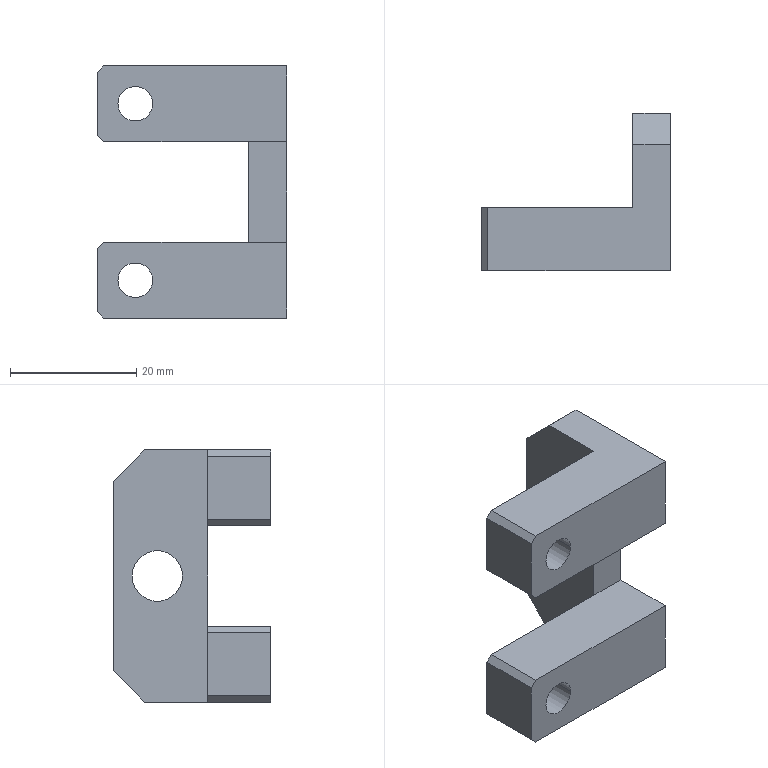Component | SolidWorks | 312981493LimitBlock-1 | 1 solid | 26 faces | box 30 x 25 x 40 mm | volume 9853 mm3 | plane 20 | cylinder 6 | commonest cylinder face diameters 5.5 x4 8 x2 | material Plain Carbon Steel
build123d program:
from build123d import *

# Parameters (mm, degrees)
SKETCH1_W            = 25
SKETCH1_H            = 40
BOSS_EXTRUDE1_DEPTH  = 30
SKETCH5_W            = 15
SKETCH5_H            = 40
CUT_EXTRUDE2_DEPTH   = 24
SKETCH9_W            = 10
SKETCH9_H            = 16
CUT_EXTRUDE4_DEPTH   = 56.902
CHAMFER2_SIZE        = 5
M5_CLEARANCE_HOLE1_D = 5.5
LPATTERN1_COUNT      = 2
LPATTERN1_PITCH      = 28
CHAMFER3_SIZE        = 1
M8_TAPPED_HOLE1_D    = 8


with BuildPart() as part:
    # Sketch1 → Boss-Extrude1 (new body)
    with BuildSketch(Plane.XY):
        with Locations((12.5, 20)):
            Rectangle(SKETCH1_W, SKETCH1_H)
    extrude(amount=BOSS_EXTRUDE1_DEPTH)

    # Sketch5 → Cut-Extrude2 (cut)
    with BuildSketch(Plane.XY.offset(30)):
        with Locations((7.5, 20)):
            Rectangle(SKETCH5_W, SKETCH5_H)
    extrude(amount=-CUT_EXTRUDE2_DEPTH, mode=Mode.SUBTRACT)

    # Sketch9 → Cut-Extrude4 (cut, through all)
    with BuildSketch(Plane.XY.offset(30)):
        with Locations((20, 20)):
            Rectangle(SKETCH9_W, SKETCH9_H)
    extrude(amount=-CUT_EXTRUDE4_DEPTH, mode=Mode.SUBTRACT)

    # Chamfer2
    chamfer2_edges = [part.edges().sort_by_distance(p)[0] for p in [
        (0, 40, 3),
        (0, 0, 3),
    ]]
    chamfer(chamfer2_edges, length=CHAMFER2_SIZE)

    # M5 Clearance Hole1 (through all)
    with Locations(Plane(origin=(15, 28.184, -31.582), x_dir=(0, 0, 1), z_dir=(-1, 0, 0))):
        with Locations((55.582, -22.184)):
            m5_clearance_hole1 = Hole(M5_CLEARANCE_HOLE1_D / 2)

    # LPattern1: M5 Clearance Hole1 ×2
    with Locations(*[(0, i * LPATTERN1_PITCH, 0) for i in range(1, LPATTERN1_COUNT)]):
        add(m5_clearance_hole1, mode=Mode.SUBTRACT)

    # Chamfer3
    chamfer3_edges = [part.edges().sort_by_distance(p)[0] for p in [
        (20, 40, 30),
        (20, 0, 30),
        (20, 28, 30),
        (20, 12, 30),
    ]]
    chamfer(chamfer3_edges, length=CHAMFER3_SIZE)

    # M8 Tapped Hole1 (through all)
    with Locations(Plane.XY.offset(6)):
        with Locations((7, 20)):
            Hole(M8_TAPPED_HOLE1_D / 2)


solid = part.part

# Placed as in the assembly
solid = solid.moved(Location((36.27, 33.768, 18.329), (90, -90, 0)))
STEP:
#1=COLOUR_RGB('',0.7922,0.8196,0.9333);
#2=FILL_AREA_STYLE_COLOUR('',#1);
#3=FILL_AREA_STYLE('',(#2));
#4=SURFACE_STYLE_FILL_AREA(#3);
#5=SURFACE_SIDE_STYLE('',(#4));
#6=SURFACE_STYLE_USAGE(.BOTH.,#5);
#7=PRESENTATION_STYLE_ASSIGNMENT((#6));
#8=CARTESIAN_POINT('',(1.428,1.211,1.509));
#9=VERTEX_POINT('',#8);
#10=CARTESIAN_POINT('',(1.428,0.8964,1.509));
#11=VERTEX_POINT('',#10);
#12=CARTESIAN_POINT('',(1.428,1.054,1.509));
#13=DIRECTION('',(-1.,-0.,-0.));
#14=DIRECTION('',(0.,-1.,0.));
#15=AXIS2_PLACEMENT_3D('',#12,#13,#14);
#16=CIRCLE('',#15,0.1575);
#17=EDGE_CURVE('',#9,#11,#16,.T.);
#18=ORIENTED_EDGE('',*,*,#17,.F.);
#19=CARTESIAN_POINT('',(1.192,1.211,1.509));
#20=VERTEX_POINT('',#19);
#21=CARTESIAN_POINT('',(1.192,1.211,1.509));
#22=DIRECTION('',(-1.,-0.,-0.));
#23=VECTOR('',#22,39.37);
#24=LINE('',#21,#23);
#25=EDGE_CURVE('',#9,#20,#24,.T.);
#26=ORIENTED_EDGE('',*,*,#25,.T.);
#27=CARTESIAN_POINT('',(1.192,0.8964,1.509));
#28=VERTEX_POINT('',#27);
#29=CARTESIAN_POINT('',(1.192,1.054,1.509));
#30=DIRECTION('',(-1.,-0.,-0.));
#31=DIRECTION('',(0.,-1.,0.));
#32=AXIS2_PLACEMENT_3D('',#29,#30,#31);
#33=CIRCLE('',#32,0.1575);
#34=EDGE_CURVE('',#20,#28,#33,.T.);
#35=ORIENTED_EDGE('',*,*,#34,.T.);
#36=CARTESIAN_POINT('',(1.192,0.8964,1.509));
#37=DIRECTION('',(-1.,-0.,-0.));
#38=VECTOR('',#37,39.37);
#39=LINE('',#36,#38);
#40=EDGE_CURVE('',#11,#28,#39,.T.);
#41=ORIENTED_EDGE('',*,*,#40,.F.);
#42=EDGE_LOOP('',(#18,#26,#35,#41));
#43=FACE_OUTER_BOUND('',#42,.T.);
#44=CARTESIAN_POINT('',(1.192,1.054,1.509));
#45=DIRECTION('',(-1.,-0.,-0.));
#46=DIRECTION('',(0.,-1.,0.));
#47=AXIS2_PLACEMENT_3D('',#44,#45,#46);
#48=CYLINDRICAL_SURFACE('',#47,0.1575);
#49=ADVANCED_FACE('',(#43),#48,.F.);
#50=CARTESIAN_POINT('',(0.5913,0.3452,2.06));
#51=VERTEX_POINT('',#50);
#52=CARTESIAN_POINT('',(0.3748,0.3452,2.06));
#53=VERTEX_POINT('',#52);
#54=CARTESIAN_POINT('',(0.4831,0.3452,2.06));
#55=DIRECTION('',(-0.,1.,-0.));
#56=DIRECTION('',(-1.,0.,0.));
#57=AXIS2_PLACEMENT_3D('',#54,#55,#56);
#58=CIRCLE('',#57,0.1083);
#59=EDGE_CURVE('',#51,#53,#58,.T.);
#60=ORIENTED_EDGE('',*,*,#59,.F.);
#61=CARTESIAN_POINT('',(0.5913,0.7389,2.06));
#62=VERTEX_POINT('',#61);
#63=CARTESIAN_POINT('',(0.5913,0.7389,2.06));
#64=DIRECTION('',(-0.,1.,-0.));
#65=VECTOR('',#64,39.37);
#66=LINE('',#63,#65);
#67=EDGE_CURVE('',#51,#62,#66,.T.);
#68=ORIENTED_EDGE('',*,*,#67,.T.);
#69=CARTESIAN_POINT('',(0.3748,0.7389,2.06));
#70=VERTEX_POINT('',#69);
#71=CARTESIAN_POINT('',(0.4831,0.7389,2.06));
#72=DIRECTION('',(-0.,1.,-0.));
#73=DIRECTION('',(-1.,0.,0.));
#74=AXIS2_PLACEMENT_3D('',#71,#72,#73);
#75=CIRCLE('',#74,0.1083);
#76=EDGE_CURVE('',#62,#70,#75,.T.);
#77=ORIENTED_EDGE('',*,*,#76,.T.);
#78=CARTESIAN_POINT('',(0.3748,0.7389,2.06));
#79=DIRECTION('',(-0.,1.,-0.));
#80=VECTOR('',#79,39.37);
#81=LINE('',#78,#80);
#82=EDGE_CURVE('',#53,#70,#81,.T.);
#83=ORIENTED_EDGE('',*,*,#82,.F.);
#84=EDGE_LOOP('',(#60,#68,#77,#83));
#85=FACE_OUTER_BOUND('',#84,.T.);
#86=CARTESIAN_POINT('',(0.4831,0.7389,2.06));
#87=DIRECTION('',(-0.,1.,-0.));
#88=DIRECTION('',(-1.,0.,0.));
#89=AXIS2_PLACEMENT_3D('',#86,#87,#88);
#90=CYLINDRICAL_SURFACE('',#89,0.1083);
#91=ADVANCED_FACE('',(#85),#90,.F.);
#92=CARTESIAN_POINT('',(0.5913,0.3452,0.9579));
#93=VERTEX_POINT('',#92);
#94=CARTESIAN_POINT('',(0.3748,0.3452,0.9579));
#95=VERTEX_POINT('',#94);
#96=CARTESIAN_POINT('',(0.4831,0.3452,0.9579));
#97=DIRECTION('',(-0.,1.,-0.));
#98=DIRECTION('',(-1.,0.,0.));
#99=AXIS2_PLACEMENT_3D('',#96,#97,#98);
#100=CIRCLE('',#99,0.1083);
#101=EDGE_CURVE('',#93,#95,#100,.T.);
#102=ORIENTED_EDGE('',*,*,#101,.F.);
#103=CARTESIAN_POINT('',(0.5913,0.7389,0.9579));
#104=VERTEX_POINT('',#103);
#105=CARTESIAN_POINT('',(0.5913,0.7389,0.9579));
#106=DIRECTION('',(-0.,1.,-0.));
#107=VECTOR('',#106,39.37);
#108=LINE('',#105,#107);
#109=EDGE_CURVE('',#93,#104,#108,.T.);
#110=ORIENTED_EDGE('',*,*,#109,.T.);
#111=CARTESIAN_POINT('',(0.3748,0.7389,0.9579));
#112=VERTEX_POINT('',#111);
#113=CARTESIAN_POINT('',(0.4831,0.7389,0.9579));
#114=DIRECTION('',(-0.,1.,-0.));
#115=DIRECTION('',(-1.,0.,0.));
#116=AXIS2_PLACEMENT_3D('',#113,#114,#115);
#117=CIRCLE('',#116,0.1083);
#118=EDGE_CURVE('',#104,#112,#117,.T.);
#119=ORIENTED_EDGE('',*,*,#118,.T.);
#120=CARTESIAN_POINT('',(0.3748,0.7389,0.9579));
#121=DIRECTION('',(-0.,1.,-0.));
#122=VECTOR('',#121,39.37);
#123=LINE('',#120,#122);
#124=EDGE_CURVE('',#95,#112,#123,.T.);
#125=ORIENTED_EDGE('',*,*,#124,.F.);
#126=EDGE_LOOP('',(#102,#110,#119,#125));
#127=FACE_OUTER_BOUND('',#126,.T.);
#128=CARTESIAN_POINT('',(0.4831,0.7389,0.9579));
#129=DIRECTION('',(-0.,1.,-0.));
#130=DIRECTION('',(-1.,0.,0.));
#131=AXIS2_PLACEMENT_3D('',#128,#129,#130);
#132=CYLINDRICAL_SURFACE('',#131,0.1083);
#133=ADVANCED_FACE('',(#127),#132,.F.);
#134=CARTESIAN_POINT('',(0.4831,0.3452,0.9579));
#135=DIRECTION('',(-0.,1.,-0.));
#136=DIRECTION('',(-1.,0.,0.));
#137=AXIS2_PLACEMENT_3D('',#134,#135,#136);
#138=CIRCLE('',#137,0.1083);
#139=EDGE_CURVE('',#95,#93,#138,.T.);
#140=ORIENTED_EDGE('',*,*,#139,.T.);
#141=ORIENTED_EDGE('',*,*,#101,.T.);
#142=EDGE_LOOP('',(#140,#141));
#143=FACE_BOUND('',#142,.T.);
#144=CARTESIAN_POINT('',(1.428,0.3452,1.194));
#145=VERTEX_POINT('',#144);
#146=CARTESIAN_POINT('',(0.2862,0.3452,1.194));
#147=VERTEX_POINT('',#146);
#148=CARTESIAN_POINT('',(1.428,0.3452,1.194));
#149=DIRECTION('',(-1.,-0.,-0.));
#150=VECTOR('',#149,39.37);
#151=LINE('',#148,#150);
#152=EDGE_CURVE('',#145,#147,#151,.T.);
#153=ORIENTED_EDGE('',*,*,#152,.T.);
#154=CARTESIAN_POINT('',(0.2469,0.3452,1.155));
#155=VERTEX_POINT('',#154);
#156=CARTESIAN_POINT('',(0.2862,0.3452,1.194));
#157=DIRECTION('',(-0.7071,-0.,-0.7071));
#158=VECTOR('',#157,39.37);
#159=LINE('',#156,#158);
#160=EDGE_CURVE('',#147,#155,#159,.T.);
#161=ORIENTED_EDGE('',*,*,#160,.T.);
#162=CARTESIAN_POINT('',(0.2469,0.3452,0.761));
#163=VERTEX_POINT('',#162);
#164=CARTESIAN_POINT('',(0.2469,0.3452,0.7216));
#165=DIRECTION('',(0.,0.,1.));
#166=VECTOR('',#165,39.37);
#167=LINE('',#164,#166);
#168=EDGE_CURVE('',#163,#155,#167,.T.);
#169=ORIENTED_EDGE('',*,*,#168,.F.);
#170=CARTESIAN_POINT('',(0.2862,0.3452,0.7216));
#171=VERTEX_POINT('',#170);
#172=CARTESIAN_POINT('',(0.2469,0.3452,0.761));
#173=DIRECTION('',(0.7071,-0.,-0.7071));
#174=VECTOR('',#173,39.37);
#175=LINE('',#172,#174);
#176=EDGE_CURVE('',#163,#171,#175,.T.);
#177=ORIENTED_EDGE('',*,*,#176,.T.);
#178=CARTESIAN_POINT('',(1.428,0.3452,0.7216));
#179=VERTEX_POINT('',#178);
#180=CARTESIAN_POINT('',(0.2469,0.3452,0.7216));
#181=DIRECTION('',(1.,0.,0.));
#182=VECTOR('',#181,39.37);
#183=LINE('',#180,#182);
#184=EDGE_CURVE('',#171,#179,#183,.T.);
#185=ORIENTED_EDGE('',*,*,#184,.T.);
#186=CARTESIAN_POINT('',(1.428,0.3452,0.7216));
#187=DIRECTION('',(0.,0.,1.));
#188=VECTOR('',#187,39.37);
#189=LINE('',#186,#188);
#190=EDGE_CURVE('',#179,#145,#189,.T.);
#191=ORIENTED_EDGE('',*,*,#190,.T.);
#192=EDGE_LOOP('',(#153,#161,#169,#177,#185,#191));
#193=FACE_OUTER_BOUND('',#192,.T.);
#194=CARTESIAN_POINT('',(0.2469,0.3452,0.7216));
#195=DIRECTION('',(-0.,1.,-0.));
#196=DIRECTION('',(-1.,-0.,-0.));
#197=AXIS2_PLACEMENT_3D('',#194,#195,#196);
#198=PLANE('',#197);
#199=ADVANCED_FACE('',(#143,#193),#198,.F.);
#200=ORIENTED_EDGE('',*,*,#168,.T.);
#201=CARTESIAN_POINT('',(0.2469,0.7389,1.155));
#202=VERTEX_POINT('',#201);
#203=CARTESIAN_POINT('',(0.2469,1.329,1.155));
#204=DIRECTION('',(-0.,1.,-0.));
#205=VECTOR('',#204,39.37);
#206=LINE('',#203,#205);
#207=EDGE_CURVE('',#155,#202,#206,.T.);
#208=ORIENTED_EDGE('',*,*,#207,.T.);
#209=CARTESIAN_POINT('',(0.2469,0.7389,0.761));
#210=VERTEX_POINT('',#209);
#211=CARTESIAN_POINT('',(0.2469,0.7389,0.7216));
#212=DIRECTION('',(0.,0.,1.));
#213=VECTOR('',#212,39.37);
#214=LINE('',#211,#213);
#215=EDGE_CURVE('',#210,#202,#214,.T.);
#216=ORIENTED_EDGE('',*,*,#215,.F.);
#217=CARTESIAN_POINT('',(0.2469,1.329,0.761));
#218=DIRECTION('',(0.,-1.,0.));
#219=VECTOR('',#218,39.37);
#220=LINE('',#217,#219);
#221=EDGE_CURVE('',#210,#163,#220,.T.);
#222=ORIENTED_EDGE('',*,*,#221,.T.);
#223=EDGE_LOOP('',(#200,#208,#216,#222));
#224=FACE_OUTER_BOUND('',#223,.T.);
#225=CARTESIAN_POINT('',(0.2469,1.329,2.296));
#226=DIRECTION('',(1.,0.,0.));
#227=DIRECTION('',(-0.,1.,-0.));
#228=AXIS2_PLACEMENT_3D('',#225,#226,#227);
#229=PLANE('',#228);
#230=ADVANCED_FACE('',(#224),#229,.F.);
#231=CARTESIAN_POINT('',(0.4831,0.7389,0.9579));
#232=DIRECTION('',(-0.,1.,-0.));
#233=DIRECTION('',(-1.,0.,0.));
#234=AXIS2_PLACEMENT_3D('',#231,#232,#233);
#235=CIRCLE('',#234,0.1083);
#236=EDGE_CURVE('',#112,#104,#235,.T.);
#237=ORIENTED_EDGE('',*,*,#236,.F.);
#238=ORIENTED_EDGE('',*,*,#118,.F.);
#239=EDGE_LOOP('',(#237,#238));
#240=FACE_BOUND('',#239,.T.);
#241=ORIENTED_EDGE('',*,*,#215,.T.);
#242=CARTESIAN_POINT('',(0.2862,0.7389,1.194));
#243=VERTEX_POINT('',#242);
#244=CARTESIAN_POINT('',(0.2862,0.7389,1.194));
#245=DIRECTION('',(0.7071,0.,0.7071));
#246=VECTOR('',#245,39.37);
#247=LINE('',#244,#246);
#248=EDGE_CURVE('',#202,#243,#247,.T.);
#249=ORIENTED_EDGE('',*,*,#248,.T.);
#250=CARTESIAN_POINT('',(1.192,0.7389,1.194));
#251=VERTEX_POINT('',#250);
#252=CARTESIAN_POINT('',(3.11,0.7389,1.194));
#253=DIRECTION('',(1.,0.,0.));
#254=VECTOR('',#253,39.37);
#255=LINE('',#252,#254);
#256=EDGE_CURVE('',#243,#251,#255,.T.);
#257=ORIENTED_EDGE('',*,*,#256,.T.);
#258=CARTESIAN_POINT('',(1.192,0.7389,0.7216));
#259=VERTEX_POINT('',#258);
#260=CARTESIAN_POINT('',(1.192,0.7389,0.7216));
#261=DIRECTION('',(0.,0.,1.));
#262=VECTOR('',#261,39.37);
#263=LINE('',#260,#262);
#264=EDGE_CURVE('',#259,#251,#263,.T.);
#265=ORIENTED_EDGE('',*,*,#264,.F.);
#266=CARTESIAN_POINT('',(0.2862,0.7389,0.7216));
#267=VERTEX_POINT('',#266);
#268=CARTESIAN_POINT('',(3.11,0.7389,0.7216));
#269=DIRECTION('',(-1.,-0.,-0.));
#270=VECTOR('',#269,39.37);
#271=LINE('',#268,#270);
#272=EDGE_CURVE('',#259,#267,#271,.T.);
#273=ORIENTED_EDGE('',*,*,#272,.T.);
#274=CARTESIAN_POINT('',(0.2469,0.7389,0.761));
#275=DIRECTION('',(-0.7071,0.,0.7071));
#276=VECTOR('',#275,39.37);
#277=LINE('',#274,#276);
#278=EDGE_CURVE('',#267,#210,#277,.T.);
#279=ORIENTED_EDGE('',*,*,#278,.T.);
#280=EDGE_LOOP('',(#241,#249,#257,#265,#273,#279));
#281=FACE_OUTER_BOUND('',#280,.T.);
#282=CARTESIAN_POINT('',(3.11,0.7389,0.7216));
#283=DIRECTION('',(0.,-1.,0.));
#284=DIRECTION('',(1.,0.,0.));
#285=AXIS2_PLACEMENT_3D('',#282,#283,#284);
#286=PLANE('',#285);
#287=ADVANCED_FACE('',(#240,#281),#286,.F.);
#288=CARTESIAN_POINT('',(1.428,1.329,2.1));
#289=VERTEX_POINT('',#288);
#290=CARTESIAN_POINT('',(1.428,1.329,0.9185));
#291=VERTEX_POINT('',#290);
#292=CARTESIAN_POINT('',(1.428,1.329,0.7216));
#293=DIRECTION('',(-0.,-0.,-1.));
#294=VECTOR('',#293,39.37);
#295=LINE('',#292,#294);
#296=EDGE_CURVE('',#289,#291,#295,.T.);
#297=ORIENTED_EDGE('',*,*,#296,.T.);
#298=CARTESIAN_POINT('',(1.192,1.329,0.9185));
#299=VERTEX_POINT('',#298);
#300=CARTESIAN_POINT('',(0.2469,1.329,0.9185));
#301=DIRECTION('',(-1.,-0.,-0.));
#302=VECTOR('',#301,39.37);
#303=LINE('',#300,#302);
#304=EDGE_CURVE('',#291,#299,#303,.T.);
#305=ORIENTED_EDGE('',*,*,#304,.T.);
#306=CARTESIAN_POINT('',(1.192,1.329,2.1));
#307=VERTEX_POINT('',#306);
#308=CARTESIAN_POINT('',(1.192,1.329,0.7216));
#309=DIRECTION('',(-0.,-0.,-1.));
#310=VECTOR('',#309,39.37);
#311=LINE('',#308,#310);
#312=EDGE_CURVE('',#307,#299,#311,.T.);
#313=ORIENTED_EDGE('',*,*,#312,.F.);
#314=CARTESIAN_POINT('',(0.2469,1.329,2.1));
#315=DIRECTION('',(1.,0.,0.));
#316=VECTOR('',#315,39.37);
#317=LINE('',#314,#316);
#318=EDGE_CURVE('',#307,#289,#317,.T.);
#319=ORIENTED_EDGE('',*,*,#318,.T.);
#320=EDGE_LOOP('',(#297,#305,#313,#319));
#321=FACE_OUTER_BOUND('',#320,.T.);
#322=CARTESIAN_POINT('',(0.2469,1.329,0.7216));
#323=DIRECTION('',(0.,-1.,0.));
#324=DIRECTION('',(1.,0.,0.));
#325=AXIS2_PLACEMENT_3D('',#322,#323,#324);
#326=PLANE('',#325);
#327=ADVANCED_FACE('',(#321),#326,.F.);
#328=ORIENTED_EDGE('',*,*,#184,.F.);
#329=CARTESIAN_POINT('',(0.2862,1.329,0.7216));
#330=DIRECTION('',(-0.,1.,-0.));
#331=VECTOR('',#330,39.37);
#332=LINE('',#329,#331);
#333=EDGE_CURVE('',#171,#267,#332,.T.);
#334=ORIENTED_EDGE('',*,*,#333,.T.);
#335=ORIENTED_EDGE('',*,*,#272,.F.);
#336=CARTESIAN_POINT('',(1.192,1.133,0.7216));
#337=VERTEX_POINT('',#336);
#338=CARTESIAN_POINT('',(1.192,0.7389,0.7216));
#339=DIRECTION('',(0.,-1.,0.));
#340=VECTOR('',#339,39.37);
#341=LINE('',#338,#340);
#342=EDGE_CURVE('',#337,#259,#341,.T.);
#343=ORIENTED_EDGE('',*,*,#342,.F.);
#344=CARTESIAN_POINT('',(1.428,1.133,0.7216));
#345=VERTEX_POINT('',#344);
#346=CARTESIAN_POINT('',(0.2469,1.133,0.7216));
#347=DIRECTION('',(1.,0.,0.));
#348=VECTOR('',#347,39.37);
#349=LINE('',#346,#348);
#350=EDGE_CURVE('',#337,#345,#349,.T.);
#351=ORIENTED_EDGE('',*,*,#350,.T.);
#352=CARTESIAN_POINT('',(1.428,1.329,0.7216));
#353=DIRECTION('',(0.,-1.,0.));
#354=VECTOR('',#353,39.37);
#355=LINE('',#352,#354);
#356=EDGE_CURVE('',#345,#179,#355,.T.);
#357=ORIENTED_EDGE('',*,*,#356,.T.);
#358=EDGE_LOOP('',(#328,#334,#335,#343,#351,#357));
#359=FACE_OUTER_BOUND('',#358,.T.);
#360=CARTESIAN_POINT('',(0.2469,1.329,0.7216));
#361=DIRECTION('',(-0.,0.,1.));
#362=DIRECTION('',(-1.,-0.,-0.));
#363=AXIS2_PLACEMENT_3D('',#360,#361,#362);
#364=PLANE('',#363);
#365=ADVANCED_FACE('',(#359),#364,.F.);
#366=CARTESIAN_POINT('',(0.4831,0.3452,2.06));
#367=DIRECTION('',(-0.,1.,-0.));
#368=DIRECTION('',(-1.,0.,0.));
#369=AXIS2_PLACEMENT_3D('',#366,#367,#368);
#370=CIRCLE('',#369,0.1083);
#371=EDGE_CURVE('',#53,#51,#370,.T.);
#372=ORIENTED_EDGE('',*,*,#371,.T.);
#373=ORIENTED_EDGE('',*,*,#59,.T.);
#374=EDGE_LOOP('',(#372,#373));
#375=FACE_BOUND('',#374,.T.);
#376=CARTESIAN_POINT('',(0.2862,0.3452,2.296));
#377=VERTEX_POINT('',#376);
#378=CARTESIAN_POINT('',(1.428,0.3452,2.296));
#379=VERTEX_POINT('',#378);
#380=CARTESIAN_POINT('',(0.2469,0.3452,2.296));
#381=DIRECTION('',(1.,0.,0.));
#382=VECTOR('',#381,39.37);
#383=LINE('',#380,#382);
#384=EDGE_CURVE('',#377,#379,#383,.T.);
#385=ORIENTED_EDGE('',*,*,#384,.F.);
#386=CARTESIAN_POINT('',(0.2469,0.3452,2.257));
#387=VERTEX_POINT('',#386);
#388=CARTESIAN_POINT('',(0.2469,0.3452,2.257));
#389=DIRECTION('',(-0.7071,-0.,-0.7071));
#390=VECTOR('',#389,39.37);
#391=LINE('',#388,#390);
#392=EDGE_CURVE('',#377,#387,#391,.T.);
#393=ORIENTED_EDGE('',*,*,#392,.T.);
#394=CARTESIAN_POINT('',(0.2469,0.3452,1.863));
#395=VERTEX_POINT('',#394);
#396=CARTESIAN_POINT('',(0.2469,0.3452,0.7216));
#397=DIRECTION('',(0.,0.,1.));
#398=VECTOR('',#397,39.37);
#399=LINE('',#396,#398);
#400=EDGE_CURVE('',#395,#387,#399,.T.);
#401=ORIENTED_EDGE('',*,*,#400,.F.);
#402=CARTESIAN_POINT('',(0.2862,0.3452,1.824));
#403=VERTEX_POINT('',#402);
#404=CARTESIAN_POINT('',(0.2862,0.3452,1.824));
#405=DIRECTION('',(0.7071,-0.,-0.7071));
#406=VECTOR('',#405,39.37);
#407=LINE('',#404,#406);
#408=EDGE_CURVE('',#395,#403,#407,.T.);
#409=ORIENTED_EDGE('',*,*,#408,.T.);
#410=CARTESIAN_POINT('',(1.428,0.3452,1.824));
#411=VERTEX_POINT('',#410);
#412=CARTESIAN_POINT('',(1.428,0.3452,1.824));
#413=DIRECTION('',(-1.,-0.,-0.));
#414=VECTOR('',#413,39.37);
#415=LINE('',#412,#414);
#416=EDGE_CURVE('',#411,#403,#415,.T.);
#417=ORIENTED_EDGE('',*,*,#416,.F.);
#418=CARTESIAN_POINT('',(1.428,0.3452,0.7216));
#419=DIRECTION('',(0.,0.,1.));
#420=VECTOR('',#419,39.37);
#421=LINE('',#418,#420);
#422=EDGE_CURVE('',#411,#379,#421,.T.);
#423=ORIENTED_EDGE('',*,*,#422,.T.);
#424=EDGE_LOOP('',(#385,#393,#401,#409,#417,#423));
#425=FACE_OUTER_BOUND('',#424,.T.);
#426=CARTESIAN_POINT('',(0.2469,0.3452,0.7216));
#427=DIRECTION('',(-0.,1.,-0.));
#428=DIRECTION('',(-1.,-0.,-0.));
#429=AXIS2_PLACEMENT_3D('',#426,#427,#428);
#430=PLANE('',#429);
#431=ADVANCED_FACE('',(#375,#425),#430,.F.);
#432=CARTESIAN_POINT('',(1.192,0.7389,2.296));
#433=VERTEX_POINT('',#432);
#434=CARTESIAN_POINT('',(0.2862,0.7389,2.296));
#435=VERTEX_POINT('',#434);
#436=CARTESIAN_POINT('',(3.11,0.7389,2.296));
#437=DIRECTION('',(-1.,-0.,-0.));
#438=VECTOR('',#437,39.37);
#439=LINE('',#436,#438);
#440=EDGE_CURVE('',#433,#435,#439,.T.);
#441=ORIENTED_EDGE('',*,*,#440,.T.);
#442=CARTESIAN_POINT('',(0.2862,1.329,2.296));
#443=DIRECTION('',(0.,-1.,0.));
#444=VECTOR('',#443,39.37);
#445=LINE('',#442,#444);
#446=EDGE_CURVE('',#435,#377,#445,.T.);
#447=ORIENTED_EDGE('',*,*,#446,.T.);
#448=ORIENTED_EDGE('',*,*,#384,.T.);
#449=CARTESIAN_POINT('',(1.428,1.133,2.296));
#450=VERTEX_POINT('',#449);
#451=CARTESIAN_POINT('',(1.428,1.329,2.296));
#452=DIRECTION('',(-0.,1.,-0.));
#453=VECTOR('',#452,39.37);
#454=LINE('',#451,#453);
#455=EDGE_CURVE('',#379,#450,#454,.T.);
#456=ORIENTED_EDGE('',*,*,#455,.T.);
#457=CARTESIAN_POINT('',(1.192,1.133,2.296));
#458=VERTEX_POINT('',#457);
#459=CARTESIAN_POINT('',(0.2469,1.133,2.296));
#460=DIRECTION('',(-1.,-0.,-0.));
#461=VECTOR('',#460,39.37);
#462=LINE('',#459,#461);
#463=EDGE_CURVE('',#450,#458,#462,.T.);
#464=ORIENTED_EDGE('',*,*,#463,.T.);
#465=CARTESIAN_POINT('',(1.192,0.7389,2.296));
#466=DIRECTION('',(-0.,1.,-0.));
#467=VECTOR('',#466,39.37);
#468=LINE('',#465,#467);
#469=EDGE_CURVE('',#433,#458,#468,.T.);
#470=ORIENTED_EDGE('',*,*,#469,.F.);
#471=EDGE_LOOP('',(#441,#447,#448,#456,#464,#470));
#472=FACE_OUTER_BOUND('',#471,.T.);
#473=CARTESIAN_POINT('',(0.2469,1.329,2.296));
#474=DIRECTION('',(0.,-0.,-1.));
#475=DIRECTION('',(1.,0.,0.));
#476=AXIS2_PLACEMENT_3D('',#473,#474,#475);
#477=PLANE('',#476);
#478=ADVANCED_FACE('',(#472),#477,.F.);
#479=ORIENTED_EDGE('',*,*,#400,.T.);
#480=CARTESIAN_POINT('',(0.2469,0.7389,2.257));
#481=VERTEX_POINT('',#480);
#482=CARTESIAN_POINT('',(0.2469,1.329,2.257));
#483=DIRECTION('',(-0.,1.,-0.));
#484=VECTOR('',#483,39.37);
#485=LINE('',#482,#484);
#486=EDGE_CURVE('',#387,#481,#485,.T.);
#487=ORIENTED_EDGE('',*,*,#486,.T.);
#488=CARTESIAN_POINT('',(0.2469,0.7389,1.863));
#489=VERTEX_POINT('',#488);
#490=CARTESIAN_POINT('',(0.2469,0.7389,0.7216));
#491=DIRECTION('',(0.,0.,1.));
#492=VECTOR('',#491,39.37);
#493=LINE('',#490,#492);
#494=EDGE_CURVE('',#489,#481,#493,.T.);
#495=ORIENTED_EDGE('',*,*,#494,.F.);
#496=CARTESIAN_POINT('',(0.2469,1.329,1.863));
#497=DIRECTION('',(0.,-1.,0.));
#498=VECTOR('',#497,39.37);
#499=LINE('',#496,#498);
#500=EDGE_CURVE('',#489,#395,#499,.T.);
#501=ORIENTED_EDGE('',*,*,#500,.T.);
#502=EDGE_LOOP('',(#479,#487,#495,#501));
#503=FACE_OUTER_BOUND('',#502,.T.);
#504=CARTESIAN_POINT('',(0.2469,1.329,2.296));
#505=DIRECTION('',(1.,0.,0.));
#506=DIRECTION('',(-0.,1.,-0.));
#507=AXIS2_PLACEMENT_3D('',#504,#505,#506);
#508=PLANE('',#507);
#509=ADVANCED_FACE('',(#503),#508,.F.);
#510=CARTESIAN_POINT('',(1.428,1.054,1.509));
#511=DIRECTION('',(-1.,-0.,-0.));
#512=DIRECTION('',(0.,-1.,0.));
#513=AXIS2_PLACEMENT_3D('',#510,#511,#512);
#514=CIRCLE('',#513,0.1575);
#515=EDGE_CURVE('',#11,#9,#514,.T.);
#516=ORIENTED_EDGE('',*,*,#515,.T.);
#517=ORIENTED_EDGE('',*,*,#17,.T.);
#518=EDGE_LOOP('',(#516,#517));
#519=FACE_BOUND('',#518,.T.);
#520=ORIENTED_EDGE('',*,*,#356,.F.);
#521=CARTESIAN_POINT('',(1.428,2.018,1.607));
#522=DIRECTION('',(-0.,0.7071,0.7071));
#523=VECTOR('',#522,39.37);
#524=LINE('',#521,#523);
#525=EDGE_CURVE('',#345,#291,#524,.T.);
#526=ORIENTED_EDGE('',*,*,#525,.T.);
#527=ORIENTED_EDGE('',*,*,#296,.F.);
#528=CARTESIAN_POINT('',(1.428,1.231,2.198));
#529=DIRECTION('',(0.,-0.7071,0.7071));
#530=VECTOR('',#529,39.37);
#531=LINE('',#528,#530);
#532=EDGE_CURVE('',#289,#450,#531,.T.);
#533=ORIENTED_EDGE('',*,*,#532,.T.);
#534=ORIENTED_EDGE('',*,*,#455,.F.);
#535=ORIENTED_EDGE('',*,*,#422,.F.);
#536=CARTESIAN_POINT('',(1.428,0.7389,1.824));
#537=VERTEX_POINT('',#536);
#538=CARTESIAN_POINT('',(1.428,0.3452,1.824));
#539=DIRECTION('',(-0.,1.,-0.));
#540=VECTOR('',#539,39.37);
#541=LINE('',#538,#540);
#542=EDGE_CURVE('',#411,#537,#541,.T.);
#543=ORIENTED_EDGE('',*,*,#542,.T.);
#544=CARTESIAN_POINT('',(1.428,0.7389,1.194));
#545=VERTEX_POINT('',#544);
#546=CARTESIAN_POINT('',(1.428,0.7389,1.824));
#547=DIRECTION('',(-0.,-0.,-1.));
#548=VECTOR('',#547,39.37);
#549=LINE('',#546,#548);
#550=EDGE_CURVE('',#537,#545,#549,.T.);
#551=ORIENTED_EDGE('',*,*,#550,.T.);
#552=CARTESIAN_POINT('',(1.428,0.3452,1.194));
#553=DIRECTION('',(0.,-1.,0.));
#554=VECTOR('',#553,39.37);
#555=LINE('',#552,#554);
#556=EDGE_CURVE('',#545,#145,#555,.T.);
#557=ORIENTED_EDGE('',*,*,#556,.T.);
#558=ORIENTED_EDGE('',*,*,#190,.F.);
#559=EDGE_LOOP('',(#520,#526,#527,#533,#534,#535,#543,#551,#557,#558));
#560=FACE_OUTER_BOUND('',#559,.T.);
#561=CARTESIAN_POINT('',(1.428,1.329,2.296));
#562=DIRECTION('',(1.,0.,0.));
#563=DIRECTION('',(-0.,1.,-0.));
#564=AXIS2_PLACEMENT_3D('',#561,#562,#563);
#565=PLANE('',#564);
#566=ADVANCED_FACE('',(#519,#560),#565,.T.);
#567=CARTESIAN_POINT('',(1.192,1.054,1.509));
#568=DIRECTION('',(-1.,-0.,-0.));
#569=DIRECTION('',(0.,-1.,0.));
#570=AXIS2_PLACEMENT_3D('',#567,#568,#569);
#571=CIRCLE('',#570,0.1575);
#572=EDGE_CURVE('',#28,#20,#571,.T.);
#573=ORIENTED_EDGE('',*,*,#572,.F.);
#574=ORIENTED_EDGE('',*,*,#34,.F.);
#575=EDGE_LOOP('',(#573,#574));
#576=FACE_BOUND('',#575,.T.);
#577=ORIENTED_EDGE('',*,*,#312,.T.);
#578=CARTESIAN_POINT('',(1.192,1.133,0.7216));
#579=DIRECTION('',(0.,-0.7071,-0.7071));
#580=VECTOR('',#579,39.37);
#581=LINE('',#578,#580);
#582=EDGE_CURVE('',#299,#337,#581,.T.);
#583=ORIENTED_EDGE('',*,*,#582,.T.);
#584=ORIENTED_EDGE('',*,*,#342,.T.);
#585=ORIENTED_EDGE('',*,*,#264,.T.);
#586=CARTESIAN_POINT('',(1.192,0.7389,1.824));
#587=VERTEX_POINT('',#586);
#588=CARTESIAN_POINT('',(1.192,0.7389,0.7216));
#589=DIRECTION('',(0.,0.,1.));
#590=VECTOR('',#589,39.37);
#591=LINE('',#588,#590);
#592=EDGE_CURVE('',#251,#587,#591,.T.);
#593=ORIENTED_EDGE('',*,*,#592,.T.);
#594=CARTESIAN_POINT('',(1.192,0.7389,0.7216));
#595=DIRECTION('',(0.,0.,1.));
#596=VECTOR('',#595,39.37);
#597=LINE('',#594,#596);
#598=EDGE_CURVE('',#587,#433,#597,.T.);
#599=ORIENTED_EDGE('',*,*,#598,.T.);
#600=ORIENTED_EDGE('',*,*,#469,.T.);
#601=CARTESIAN_POINT('',(1.192,1.329,2.1));
#602=DIRECTION('',(-0.,0.7071,-0.7071));
#603=VECTOR('',#602,39.37);
#604=LINE('',#601,#603);
#605=EDGE_CURVE('',#458,#307,#604,.T.);
#606=ORIENTED_EDGE('',*,*,#605,.T.);
#607=EDGE_LOOP('',(#577,#583,#584,#585,#593,#599,#600,#606));
#608=FACE_OUTER_BOUND('',#607,.T.);
#609=CARTESIAN_POINT('',(1.192,1.329,2.296));
#610=DIRECTION('',(1.,0.,0.));
#611=DIRECTION('',(-0.,1.,-0.));
#612=AXIS2_PLACEMENT_3D('',#609,#610,#611);
#613=PLANE('',#612);
#614=ADVANCED_FACE('',(#576,#608),#613,.F.);
#615=CARTESIAN_POINT('',(0.4831,0.7389,2.06));
#616=DIRECTION('',(-0.,1.,-0.));
#617=DIRECTION('',(-1.,0.,0.));
#618=AXIS2_PLACEMENT_3D('',#615,#616,#617);
#619=CIRCLE('',#618,0.1083);
#620=EDGE_CURVE('',#70,#62,#619,.T.);
#621=ORIENTED_EDGE('',*,*,#620,.F.);
#622=ORIENTED_EDGE('',*,*,#76,.F.);
#623=EDGE_LOOP('',(#621,#622));
#624=FACE_BOUND('',#623,.T.);
#625=ORIENTED_EDGE('',*,*,#494,.T.);
#626=CARTESIAN_POINT('',(0.2469,0.7389,2.257));
#627=DIRECTION('',(0.7071,0.,0.7071));
#628=VECTOR('',#627,39.37);
#629=LINE('',#626,#628);
#630=EDGE_CURVE('',#481,#435,#629,.T.);
#631=ORIENTED_EDGE('',*,*,#630,.T.);
#632=ORIENTED_EDGE('',*,*,#440,.F.);
#633=ORIENTED_EDGE('',*,*,#598,.F.);
#634=CARTESIAN_POINT('',(0.2862,0.7389,1.824));
#635=VERTEX_POINT('',#634);
#636=CARTESIAN_POINT('',(3.11,0.7389,1.824));
#637=DIRECTION('',(-1.,-0.,-0.));
#638=VECTOR('',#637,39.37);
#639=LINE('',#636,#638);
#640=EDGE_CURVE('',#587,#635,#639,.T.);
#641=ORIENTED_EDGE('',*,*,#640,.T.);
#642=CARTESIAN_POINT('',(0.2862,0.7389,1.824));
#643=DIRECTION('',(-0.7071,0.,0.7071));
#644=VECTOR('',#643,39.37);
#645=LINE('',#642,#644);
#646=EDGE_CURVE('',#635,#489,#645,.T.);
#647=ORIENTED_EDGE('',*,*,#646,.T.);
#648=EDGE_LOOP('',(#625,#631,#632,#633,#641,#647));
#649=FACE_OUTER_BOUND('',#648,.T.);
#650=CARTESIAN_POINT('',(3.11,0.7389,0.7216));
#651=DIRECTION('',(0.,-1.,0.));
#652=DIRECTION('',(1.,0.,0.));
#653=AXIS2_PLACEMENT_3D('',#650,#651,#652);
#654=PLANE('',#653);
#655=ADVANCED_FACE('',(#624,#649),#654,.F.);
#656=CARTESIAN_POINT('',(1.428,0.7389,1.194));
#657=DIRECTION('',(-1.,-0.,-0.));
#658=VECTOR('',#657,39.37);
#659=LINE('',#656,#658);
#660=EDGE_CURVE('',#545,#251,#659,.T.);
#661=ORIENTED_EDGE('',*,*,#660,.F.);
#662=ORIENTED_EDGE('',*,*,#550,.F.);
#663=CARTESIAN_POINT('',(1.428,0.7389,1.824));
#664=DIRECTION('',(-1.,-0.,-0.));
#665=VECTOR('',#664,39.37);
#666=LINE('',#663,#665);
#667=EDGE_CURVE('',#537,#587,#666,.T.);
#668=ORIENTED_EDGE('',*,*,#667,.T.);
#669=ORIENTED_EDGE('',*,*,#592,.F.);
#670=EDGE_LOOP('',(#661,#662,#668,#669));
#671=FACE_OUTER_BOUND('',#670,.T.);
#672=CARTESIAN_POINT('',(1.428,0.7389,1.824));
#673=DIRECTION('',(-0.,1.,-0.));
#674=DIRECTION('',(-1.,-0.,-0.));
#675=AXIS2_PLACEMENT_3D('',#672,#673,#674);
#676=PLANE('',#675);
#677=ADVANCED_FACE('',(#671),#676,.F.);
#678=ORIENTED_EDGE('',*,*,#256,.F.);
#679=CARTESIAN_POINT('',(0.2862,0.3452,1.194));
#680=DIRECTION('',(0.,-1.,0.));
#681=VECTOR('',#680,39.37);
#682=LINE('',#679,#681);
#683=EDGE_CURVE('',#243,#147,#682,.T.);
#684=ORIENTED_EDGE('',*,*,#683,.T.);
#685=ORIENTED_EDGE('',*,*,#152,.F.);
#686=ORIENTED_EDGE('',*,*,#556,.F.);
#687=ORIENTED_EDGE('',*,*,#660,.T.);
#688=EDGE_LOOP('',(#678,#684,#685,#686,#687));
#689=FACE_OUTER_BOUND('',#688,.T.);
#690=CARTESIAN_POINT('',(1.428,0.3452,1.194));
#691=DIRECTION('',(-0.,-0.,-1.));
#692=DIRECTION('',(0.,-1.,0.));
#693=AXIS2_PLACEMENT_3D('',#690,#691,#692);
#694=PLANE('',#693);
#695=ADVANCED_FACE('',(#689),#694,.F.);
#696=ORIENTED_EDGE('',*,*,#416,.T.);
#697=CARTESIAN_POINT('',(0.2862,0.3452,1.824));
#698=DIRECTION('',(-0.,1.,-0.));
#699=VECTOR('',#698,39.37);
#700=LINE('',#697,#699);
#701=EDGE_CURVE('',#403,#635,#700,.T.);
#702=ORIENTED_EDGE('',*,*,#701,.T.);
#703=ORIENTED_EDGE('',*,*,#640,.F.);
#704=ORIENTED_EDGE('',*,*,#667,.F.);
#705=ORIENTED_EDGE('',*,*,#542,.F.);
#706=EDGE_LOOP('',(#696,#702,#703,#704,#705));
#707=FACE_OUTER_BOUND('',#706,.T.);
#708=CARTESIAN_POINT('',(1.428,0.3452,1.824));
#709=DIRECTION('',(0.,0.,1.));
#710=DIRECTION('',(-0.,1.,-0.));
#711=AXIS2_PLACEMENT_3D('',#708,#709,#710);
#712=PLANE('',#711);
#713=ADVANCED_FACE('',(#707),#712,.F.);
#714=ORIENTED_EDGE('',*,*,#582,.F.);
#715=ORIENTED_EDGE('',*,*,#304,.F.);
#716=ORIENTED_EDGE('',*,*,#525,.F.);
#717=ORIENTED_EDGE('',*,*,#350,.F.);
#718=EDGE_LOOP('',(#714,#715,#716,#717));
#719=FACE_OUTER_BOUND('',#718,.T.);
#720=CARTESIAN_POINT('',(0.2469,1.133,0.7216));
#721=DIRECTION('',(0.,-0.7071,0.7071));
#722=DIRECTION('',(-0.,0.7071,0.7071));
#723=AXIS2_PLACEMENT_3D('',#720,#721,#722);
#724=PLANE('',#723);
#725=ADVANCED_FACE('',(#719),#724,.F.);
#726=ORIENTED_EDGE('',*,*,#605,.F.);
#727=ORIENTED_EDGE('',*,*,#463,.F.);
#728=ORIENTED_EDGE('',*,*,#532,.F.);
#729=ORIENTED_EDGE('',*,*,#318,.F.);
#730=EDGE_LOOP('',(#726,#727,#728,#729));
#731=FACE_OUTER_BOUND('',#730,.T.);
#732=CARTESIAN_POINT('',(0.2469,1.329,2.1));
#733=DIRECTION('',(0.,-0.7071,-0.7071));
#734=DIRECTION('',(0.,-0.7071,0.7071));
#735=AXIS2_PLACEMENT_3D('',#732,#733,#734);
#736=PLANE('',#735);
#737=ADVANCED_FACE('',(#731),#736,.F.);
#738=ORIENTED_EDGE('',*,*,#109,.F.);
#739=ORIENTED_EDGE('',*,*,#139,.F.);
#740=ORIENTED_EDGE('',*,*,#124,.T.);
#741=ORIENTED_EDGE('',*,*,#236,.T.);
#742=EDGE_LOOP('',(#738,#739,#740,#741));
#743=FACE_OUTER_BOUND('',#742,.T.);
#744=CARTESIAN_POINT('',(0.4831,0.7389,0.9579));
#745=DIRECTION('',(-0.,1.,-0.));
#746=DIRECTION('',(-1.,0.,0.));
#747=AXIS2_PLACEMENT_3D('',#744,#745,#746);
#748=CYLINDRICAL_SURFACE('',#747,0.1083);
#749=ADVANCED_FACE('',(#743),#748,.F.);
#750=ORIENTED_EDGE('',*,*,#67,.F.);
#751=ORIENTED_EDGE('',*,*,#371,.F.);
#752=ORIENTED_EDGE('',*,*,#82,.T.);
#753=ORIENTED_EDGE('',*,*,#620,.T.);
#754=EDGE_LOOP('',(#750,#751,#752,#753));
#755=FACE_OUTER_BOUND('',#754,.T.);
#756=CARTESIAN_POINT('',(0.4831,0.7389,2.06));
#757=DIRECTION('',(-0.,1.,-0.));
#758=DIRECTION('',(-1.,0.,0.));
#759=AXIS2_PLACEMENT_3D('',#756,#757,#758);
#760=CYLINDRICAL_SURFACE('',#759,0.1083);
#761=ADVANCED_FACE('',(#755),#760,.F.);
#762=ORIENTED_EDGE('',*,*,#392,.F.);
#763=ORIENTED_EDGE('',*,*,#446,.F.);
#764=ORIENTED_EDGE('',*,*,#630,.F.);
#765=ORIENTED_EDGE('',*,*,#486,.F.);
#766=EDGE_LOOP('',(#762,#763,#764,#765));
#767=FACE_OUTER_BOUND('',#766,.T.);
#768=CARTESIAN_POINT('',(0.2469,1.329,2.257));
#769=DIRECTION('',(0.7071,-0.,-0.7071));
#770=DIRECTION('',(0.7071,0.,0.7071));
#771=AXIS2_PLACEMENT_3D('',#768,#769,#770);
#772=PLANE('',#771);
#773=ADVANCED_FACE('',(#767),#772,.F.);
#774=ORIENTED_EDGE('',*,*,#408,.F.);
#775=ORIENTED_EDGE('',*,*,#500,.F.);
#776=ORIENTED_EDGE('',*,*,#646,.F.);
#777=ORIENTED_EDGE('',*,*,#701,.F.);
#778=EDGE_LOOP('',(#774,#775,#776,#777));
#779=FACE_OUTER_BOUND('',#778,.T.);
#780=CARTESIAN_POINT('',(0.2862,0.3452,1.824));
#781=DIRECTION('',(0.7071,0.,0.7071));
#782=DIRECTION('',(-0.7071,0.,0.7071));
#783=AXIS2_PLACEMENT_3D('',#780,#781,#782);
#784=PLANE('',#783);
#785=ADVANCED_FACE('',(#779),#784,.F.);
#786=ORIENTED_EDGE('',*,*,#248,.F.);
#787=ORIENTED_EDGE('',*,*,#207,.F.);
#788=ORIENTED_EDGE('',*,*,#160,.F.);
#789=ORIENTED_EDGE('',*,*,#683,.F.);
#790=EDGE_LOOP('',(#786,#787,#788,#789));
#791=FACE_OUTER_BOUND('',#790,.T.);
#792=CARTESIAN_POINT('',(0.2862,0.3452,1.194));
#793=DIRECTION('',(0.7071,-0.,-0.7071));
#794=DIRECTION('',(0.7071,0.,0.7071));
#795=AXIS2_PLACEMENT_3D('',#792,#793,#794);
#796=PLANE('',#795);
#797=ADVANCED_FACE('',(#791),#796,.F.);
#798=ORIENTED_EDGE('',*,*,#278,.F.);
#799=ORIENTED_EDGE('',*,*,#333,.F.);
#800=ORIENTED_EDGE('',*,*,#176,.F.);
#801=ORIENTED_EDGE('',*,*,#221,.F.);
#802=EDGE_LOOP('',(#798,#799,#800,#801));
#803=FACE_OUTER_BOUND('',#802,.T.);
#804=CARTESIAN_POINT('',(0.2469,1.329,0.761));
#805=DIRECTION('',(0.7071,0.,0.7071));
#806=DIRECTION('',(-0.7071,0.,0.7071));
#807=AXIS2_PLACEMENT_3D('',#804,#805,#806);
#808=PLANE('',#807);
#809=ADVANCED_FACE('',(#803),#808,.F.);
#810=ORIENTED_EDGE('',*,*,#25,.F.);
#811=ORIENTED_EDGE('',*,*,#515,.F.);
#812=ORIENTED_EDGE('',*,*,#40,.T.);
#813=ORIENTED_EDGE('',*,*,#572,.T.);
#814=EDGE_LOOP('',(#810,#811,#812,#813));
#815=FACE_OUTER_BOUND('',#814,.T.);
#816=CARTESIAN_POINT('',(1.192,1.054,1.509));
#817=DIRECTION('',(-1.,-0.,-0.));
#818=DIRECTION('',(0.,-1.,0.));
#819=AXIS2_PLACEMENT_3D('',#816,#817,#818);
#820=CYLINDRICAL_SURFACE('',#819,0.1575);
#821=ADVANCED_FACE('',(#815),#820,.F.);
#822=CLOSED_SHELL('',(#49,#91,#133,#199,#230,#287,#327,#365,#431,#478,#509,#566,#614,#655,#677,#695,#713,#725,#737,#749,#761,#773,#785,#797,#809,#821));
#823=MANIFOLD_SOLID_BREP('',#822);
#824=STYLED_ITEM('',(#7),#823);
#825=(LENGTH_UNIT()NAMED_UNIT(*)SI_UNIT($,.METRE.));
#826=LENGTH_MEASURE_WITH_UNIT(LENGTH_MEASURE(0.0254),#825);
#827=DIMENSIONAL_EXPONENTS(1.,0.,0.,0.,0.,0.,0.);
#828=(CONVERSION_BASED_UNIT('',#826)LENGTH_UNIT()NAMED_UNIT(#827));
#829=UNCERTAINTY_MEASURE_WITH_UNIT(LENGTH_MEASURE(0.00001),#828,'','');
#830=(NAMED_UNIT(*)PLANE_ANGLE_UNIT()SI_UNIT($,.RADIAN.));
#831=(NAMED_UNIT(*)SI_UNIT($,.STERADIAN.)SOLID_ANGLE_UNIT());
#832=(GEOMETRIC_REPRESENTATION_CONTEXT(3)GLOBAL_UNCERTAINTY_ASSIGNED_CONTEXT((#829))GLOBAL_UNIT_ASSIGNED_CONTEXT((#828,#830,#831))REPRESENTATION_CONTEXT('',''));
#833=MECHANICAL_DESIGN_GEOMETRIC_PRESENTATION_REPRESENTATION('',(#824),#832);
#834=PRESENTATION_LAYER_ASSIGNMENT('','',(#824));
#835=CARTESIAN_POINT('',(0.,0.,0.));
#836=DIRECTION('',(0.,0.,1.));
#837=DIRECTION('',(1.,0.,0.));
#838=AXIS2_PLACEMENT_3D('',#835,#836,#837);
#839=(LENGTH_UNIT()NAMED_UNIT(*)SI_UNIT($,.METRE.));
#840=LENGTH_MEASURE_WITH_UNIT(LENGTH_MEASURE(0.0254),#839);
#841=DIMENSIONAL_EXPONENTS(1.,0.,0.,0.,0.,0.,0.);
#842=(CONVERSION_BASED_UNIT('',#840)LENGTH_UNIT()NAMED_UNIT(#841));
#843=UNCERTAINTY_MEASURE_WITH_UNIT(LENGTH_MEASURE(0.00001),#842,'','');
#844=(NAMED_UNIT(*)PLANE_ANGLE_UNIT()SI_UNIT($,.RADIAN.));
#845=(NAMED_UNIT(*)SI_UNIT($,.STERADIAN.)SOLID_ANGLE_UNIT());
#846=(GEOMETRIC_REPRESENTATION_CONTEXT(3)GLOBAL_UNCERTAINTY_ASSIGNED_CONTEXT((#843))GLOBAL_UNIT_ASSIGNED_CONTEXT((#842,#844,#845))REPRESENTATION_CONTEXT('',''));
#847=ADVANCED_BREP_SHAPE_REPRESENTATION('',(#823,#838),#846);